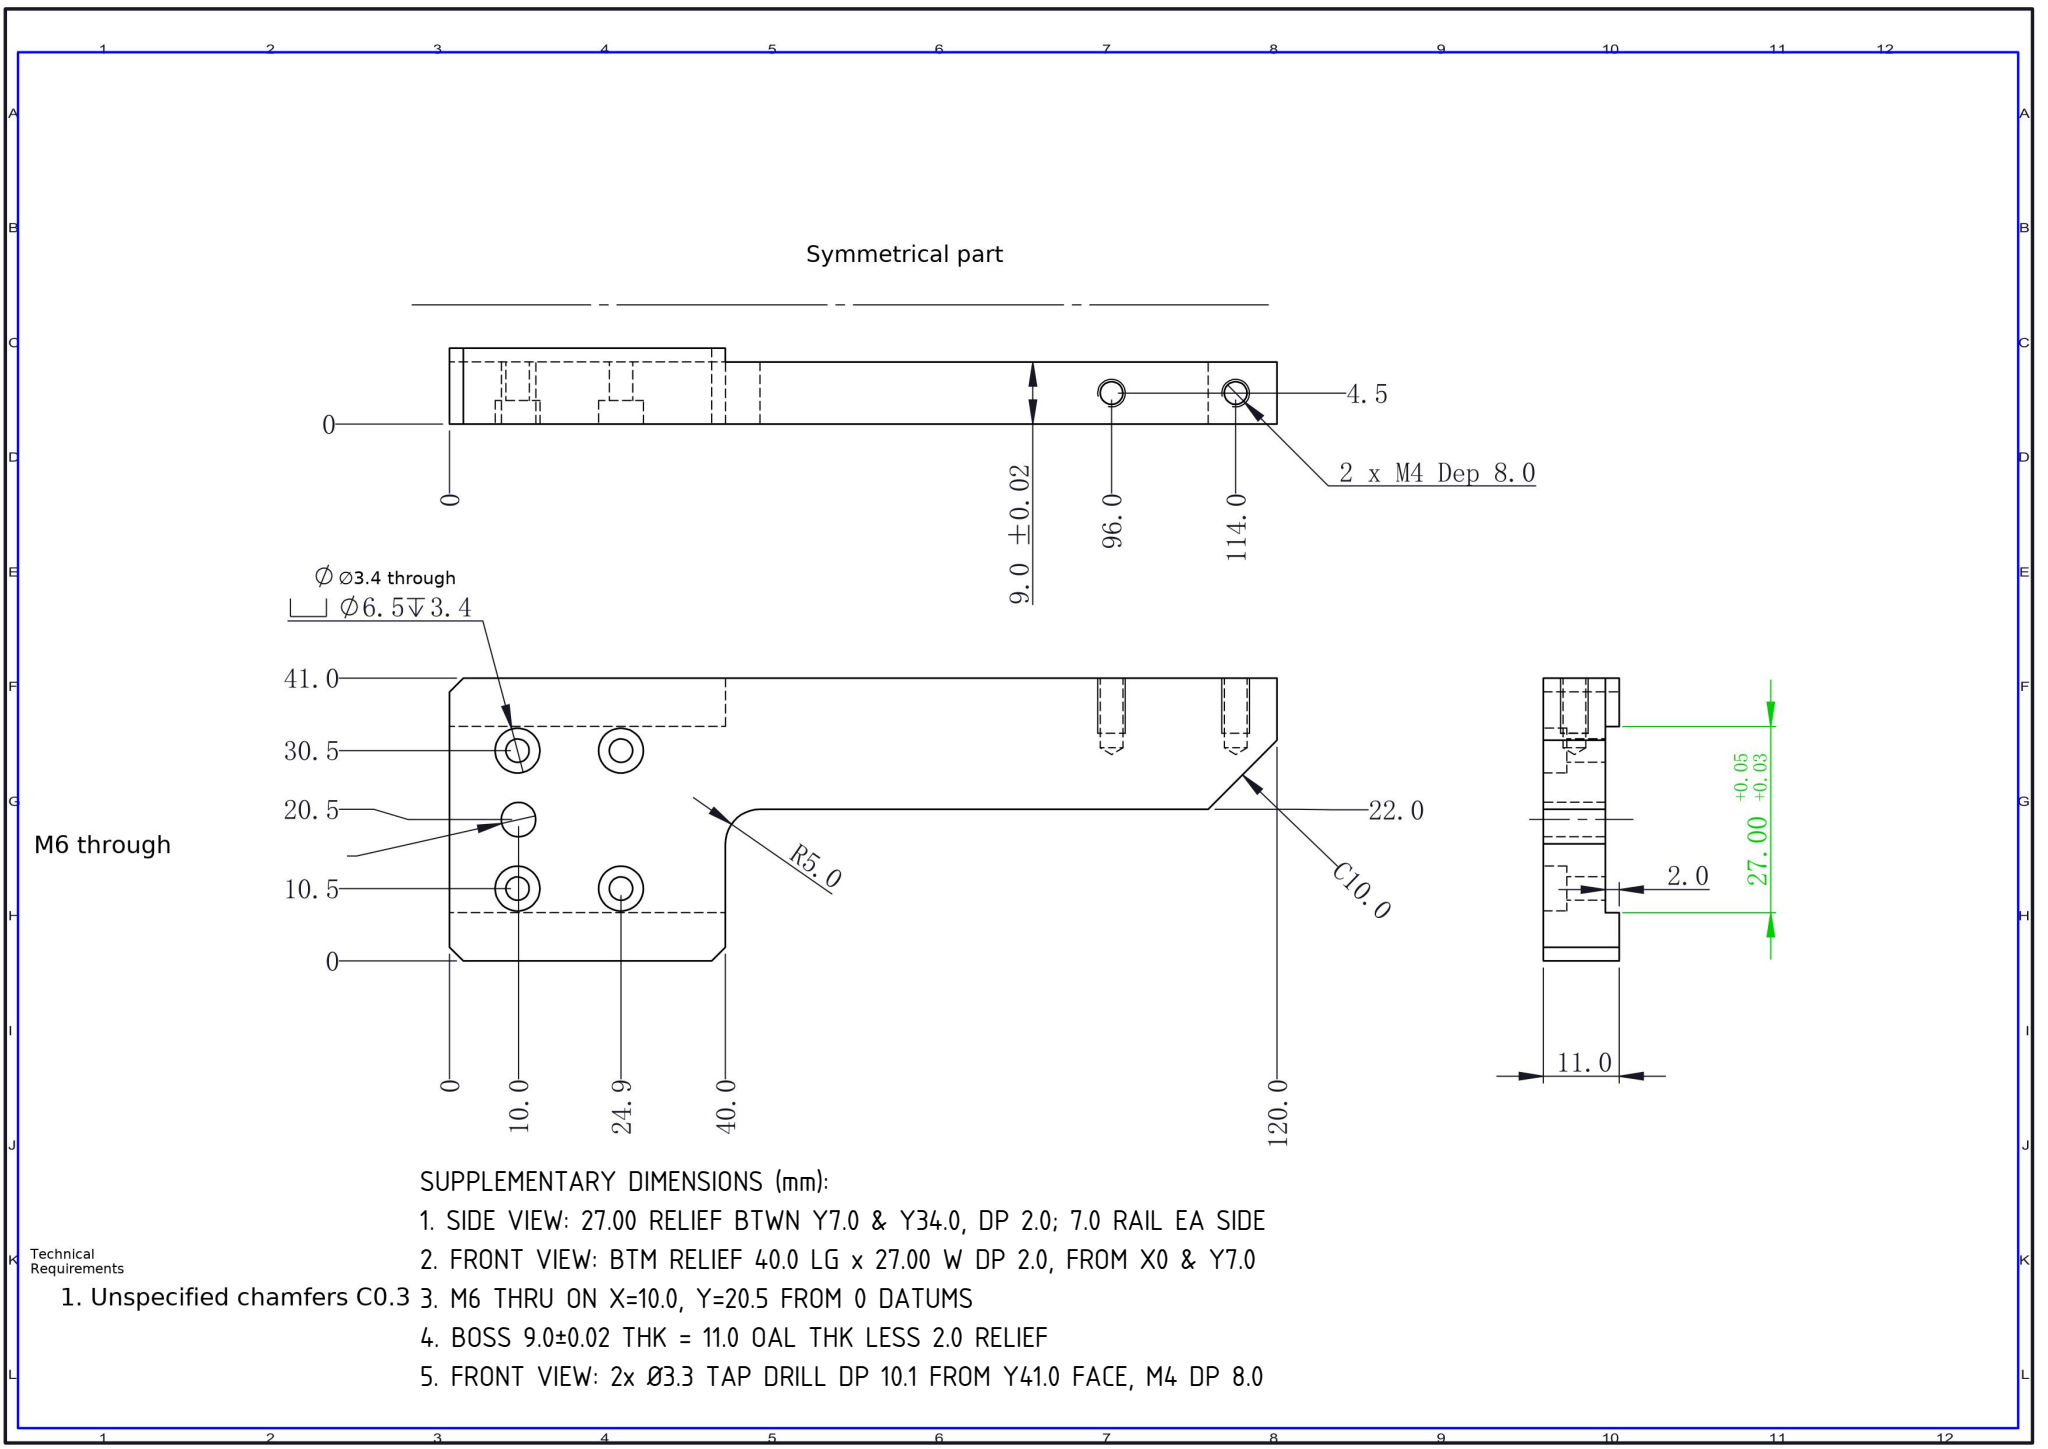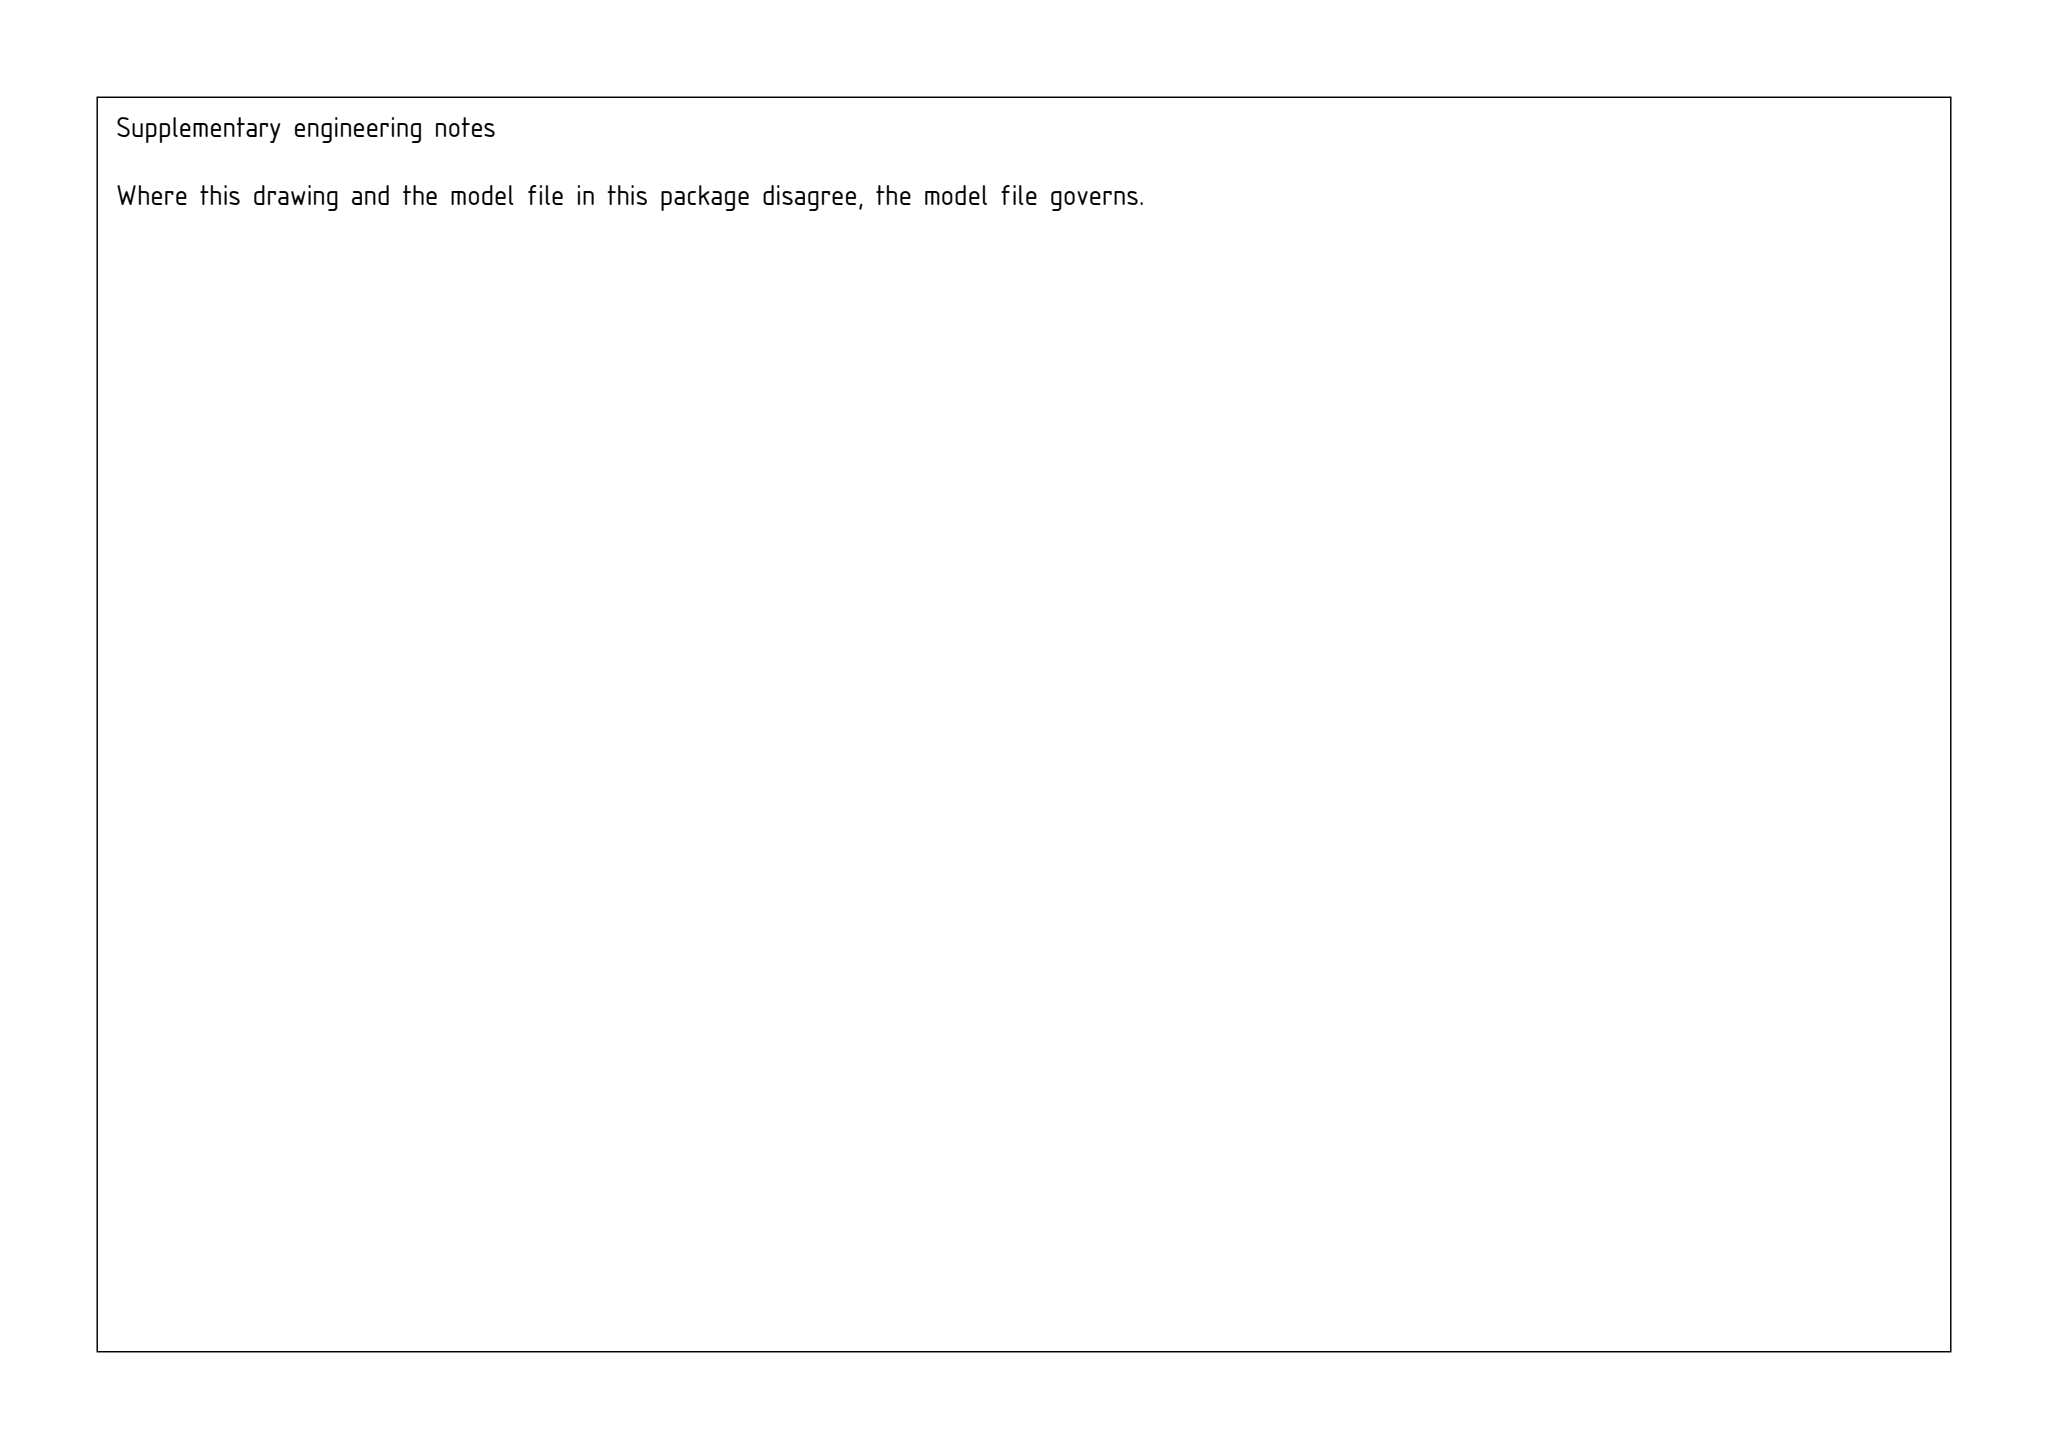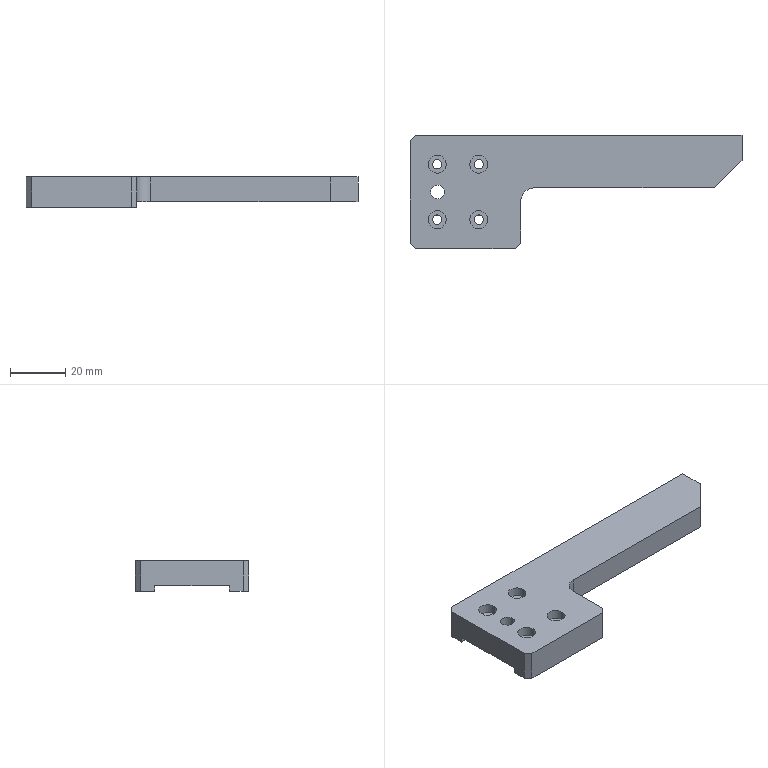Part | SolidWorks | mm | 1 solid | 48 faces | box 120 x 41 x 11 mm | volume 28082 mm3 | cylinder 23 | plane 21 | cone 4 | commonest cylinder face diameters 6.5 x8 3.4 x8 3.3 x4 5 x2 10 x1